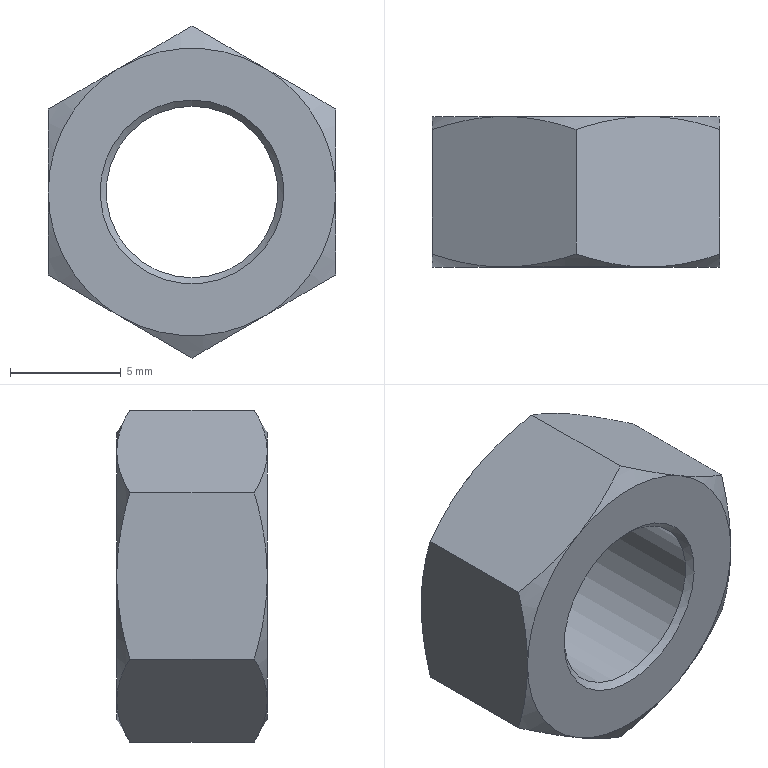Component | NX | NUT_M8 | 1 solid | 23 faces | volume 667 mm3 | cone 14 | plane 8 | cylinder 1 | commonest cylinder face diameters 7.76 x1